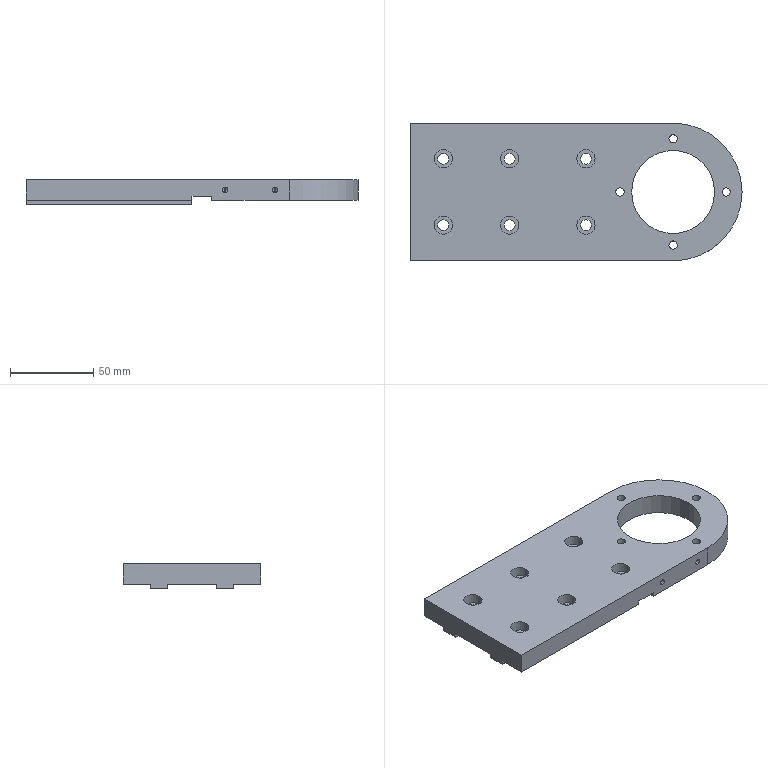Component | SolidWorks | Q1-A12-S21-Q1C.SLDASQ-1_Q1-A12-S21-Q1C-01B-1 | 1 solid | 74 faces | box 200 x 83 x 15 mm | volume 169951 mm3 | cylinder 43 | plane 23 | cone 8 | commonest cylinder face diameters 11 x12 6.6 x12 3.3 x8 5 x8 50.01 x2 83 x1 | material S-45C
build123d program:
from build123d import *

# Parameters (mm, degrees)
SKETCH1_W                                            = 200
SKETCH1_H                                            = 83
BOSS_EXTRUDE1_DEPTH                                  = 15
SKETCH2_W                                            = 2.5
SKETCH2_H                                            = 16.5
SKETCH2_H_2                                          = 30
CUT_EXTRUDE1_DEPTH                                   = 205.81
CUT_EXTRUDE2_DEPTH                                   = 110.303
SKETCH4_W                                            = 12
SKETCH4_H                                            = 5
CUT_EXTRUDE3_DEPTH                                   = 131.82
F_25_5_25_5_DIAMETER_HOLE3_D                         = 50.01
SKETCH7_W                                            = 88
SKETCH7_H                                            = 2.5
CUT_EXTRUDE4_DEPTH                                   = 131.82
CYLINDRICAL_COUNTERSUNK_HOLE_FOR_M6_SOCK_D           = 6.6
CYLINDRICAL_COUNTERSUNK_HOLE_FOR_M6_SOCK_CBORE_D     = 11
CYLINDRICAL_COUNTERSUNK_HOLE_FOR_M6_SOCK_CBORE_DEPTH = 6
M6X1_0_TAPPED_HOLE1_D                                = 5
M4X0_7_TAPPED_HOLE1_D                                = 3.3
M4X0_7_TAPPED_HOLE1_DEPTH                            = 10.1
M4X0_7_TAPPED_HOLE1_TIP                              = 0.9914
M4X0_7_TAPPED_HOLE2_D                                = 3.3
M4X0_7_TAPPED_HOLE2_DEPTH                            = 10.1
M4X0_7_TAPPED_HOLE2_TIP                              = 0.9914


with BuildPart() as part:
    # Sketch1 → Boss-Extrude1 (new body)
    with BuildSketch(Plane.XY):
        Rectangle(SKETCH1_W, SKETCH1_H)
    extrude(amount=BOSS_EXTRUDE1_DEPTH)

    # Sketch2 → Cut-Extrude1 (cut, through all)
    with BuildSketch(Plane(origin=(100, 0, 0), x_dir=(0, 0, -1), z_dir=(1, 0, 0))):
        with Locations((-1.25, 33.25)):
            Rectangle(SKETCH2_W, SKETCH2_H)
        with Locations((-1.25, 0)):
            Rectangle(SKETCH2_W, SKETCH2_H_2)
        with Locations((-1.25, -33.25)):
            Rectangle(SKETCH2_W, SKETCH2_H)
    extrude(amount=-CUT_EXTRUDE1_DEPTH, mode=Mode.SUBTRACT)

    # Sketch3 → Cut-Extrude2 (cut, through all)
    with BuildSketch(Plane.XY.offset(15)):
        with BuildLine():
            ThreePointArc((-100, 0), (-87.845, 29.345), (-58.5, 41.5))
            Line((-58.5, 41.5), (-100, 41.5))
            Line((-100, 41.5), (-100, 0))
        make_face()
        with BuildLine():
            ThreePointArc((-58.5, -41.5), (-87.845, -29.345), (-100, 0))
            Line((-100, 0), (-100, -41.5))
            Line((-100, -41.5), (-58.5, -41.5))
        make_face()
    extrude(amount=-CUT_EXTRUDE2_DEPTH, mode=Mode.SUBTRACT)

    # Sketch4 → Cut-Extrude3 (cut, through all)
    with BuildSketch(Plane(origin=(0, 41.5, 0), x_dir=(1, 0, 0), z_dir=(0, 1, 0))):
        with Locations((-6, -2.5)):
            Rectangle(SKETCH4_W, SKETCH4_H)
    extrude(amount=-CUT_EXTRUDE3_DEPTH, mode=Mode.SUBTRACT)

    # 25.5 _25.5_ Diameter Hole3 (through all)
    with Locations(Plane.XY.offset(15)):
        with Locations((-58.5, 0)):
            Hole(F_25_5_25_5_DIAMETER_HOLE3_D / 2)

    # Sketch7 → Cut-Extrude4 (cut, through all)
    with BuildSketch(Plane(origin=(0, 41.5, 0), x_dir=(1, 0, 0), z_dir=(0, 1, 0))):
        with Locations((-56, -1.25)):
            Rectangle(SKETCH7_W, SKETCH7_H)
    extrude(amount=-CUT_EXTRUDE4_DEPTH, mode=Mode.SUBTRACT)

    # Cylindrical Countersunk Hole for M6 Sock (through all)
    with Locations(Plane.XY.offset(15)):
        with Locations((-6, 20), (-6, -20), (80, 20), (40, 20), (80, -20), (40, -20)):
            CounterBoreHole(CYLINDRICAL_COUNTERSUNK_HOLE_FOR_M6_SOCK_D / 2, CYLINDRICAL_COUNTERSUNK_HOLE_FOR_M6_SOCK_CBORE_D / 2, CYLINDRICAL_COUNTERSUNK_HOLE_FOR_M6_SOCK_CBORE_DEPTH)

    # M6x1.0 Tapped Hole1 (through all)
    with Locations(Plane.XY.offset(15)):
        with Locations((-58.5, 32), (-90.5, 0), (-58.5, -32), (-26.5, 0)):
            Hole(M6X1_0_TAPPED_HOLE1_D / 2)

    # M4x0.7 Tapped Hole1
    with Locations(Plane(origin=(0, 41.5, 0), x_dir=(1, 0, 0), z_dir=(0, 1, 0))):
        with Locations((-50, -8.75), (-20, -8.75)):
            Hole(M4X0_7_TAPPED_HOLE1_D / 2, depth=M4X0_7_TAPPED_HOLE1_DEPTH)
            with Locations((0, 0, -(M4X0_7_TAPPED_HOLE1_DEPTH + M4X0_7_TAPPED_HOLE1_TIP / 2))):  # 118° drill point
                Cone(0, M4X0_7_TAPPED_HOLE1_D / 2, M4X0_7_TAPPED_HOLE1_TIP, mode=Mode.SUBTRACT)

    # M4x0.7 Tapped Hole2
    with Locations(Plane(origin=(0, -41.5, 0), x_dir=(-1, 0, 0), z_dir=(0, -1, 0))):
        with Locations((50, -8.75), (20, -8.75)):
            Hole(M4X0_7_TAPPED_HOLE2_D / 2, depth=M4X0_7_TAPPED_HOLE2_DEPTH)
            with Locations((0, 0, -(M4X0_7_TAPPED_HOLE2_DEPTH + M4X0_7_TAPPED_HOLE2_TIP / 2))):  # 118° drill point
                Cone(0, M4X0_7_TAPPED_HOLE2_D / 2, M4X0_7_TAPPED_HOLE2_TIP, mode=Mode.SUBTRACT)


solid = part.part

# Placed as in the assembly
solid = solid.moved(Location((2089.5, 0, 147.5), (0, 0, 180)))